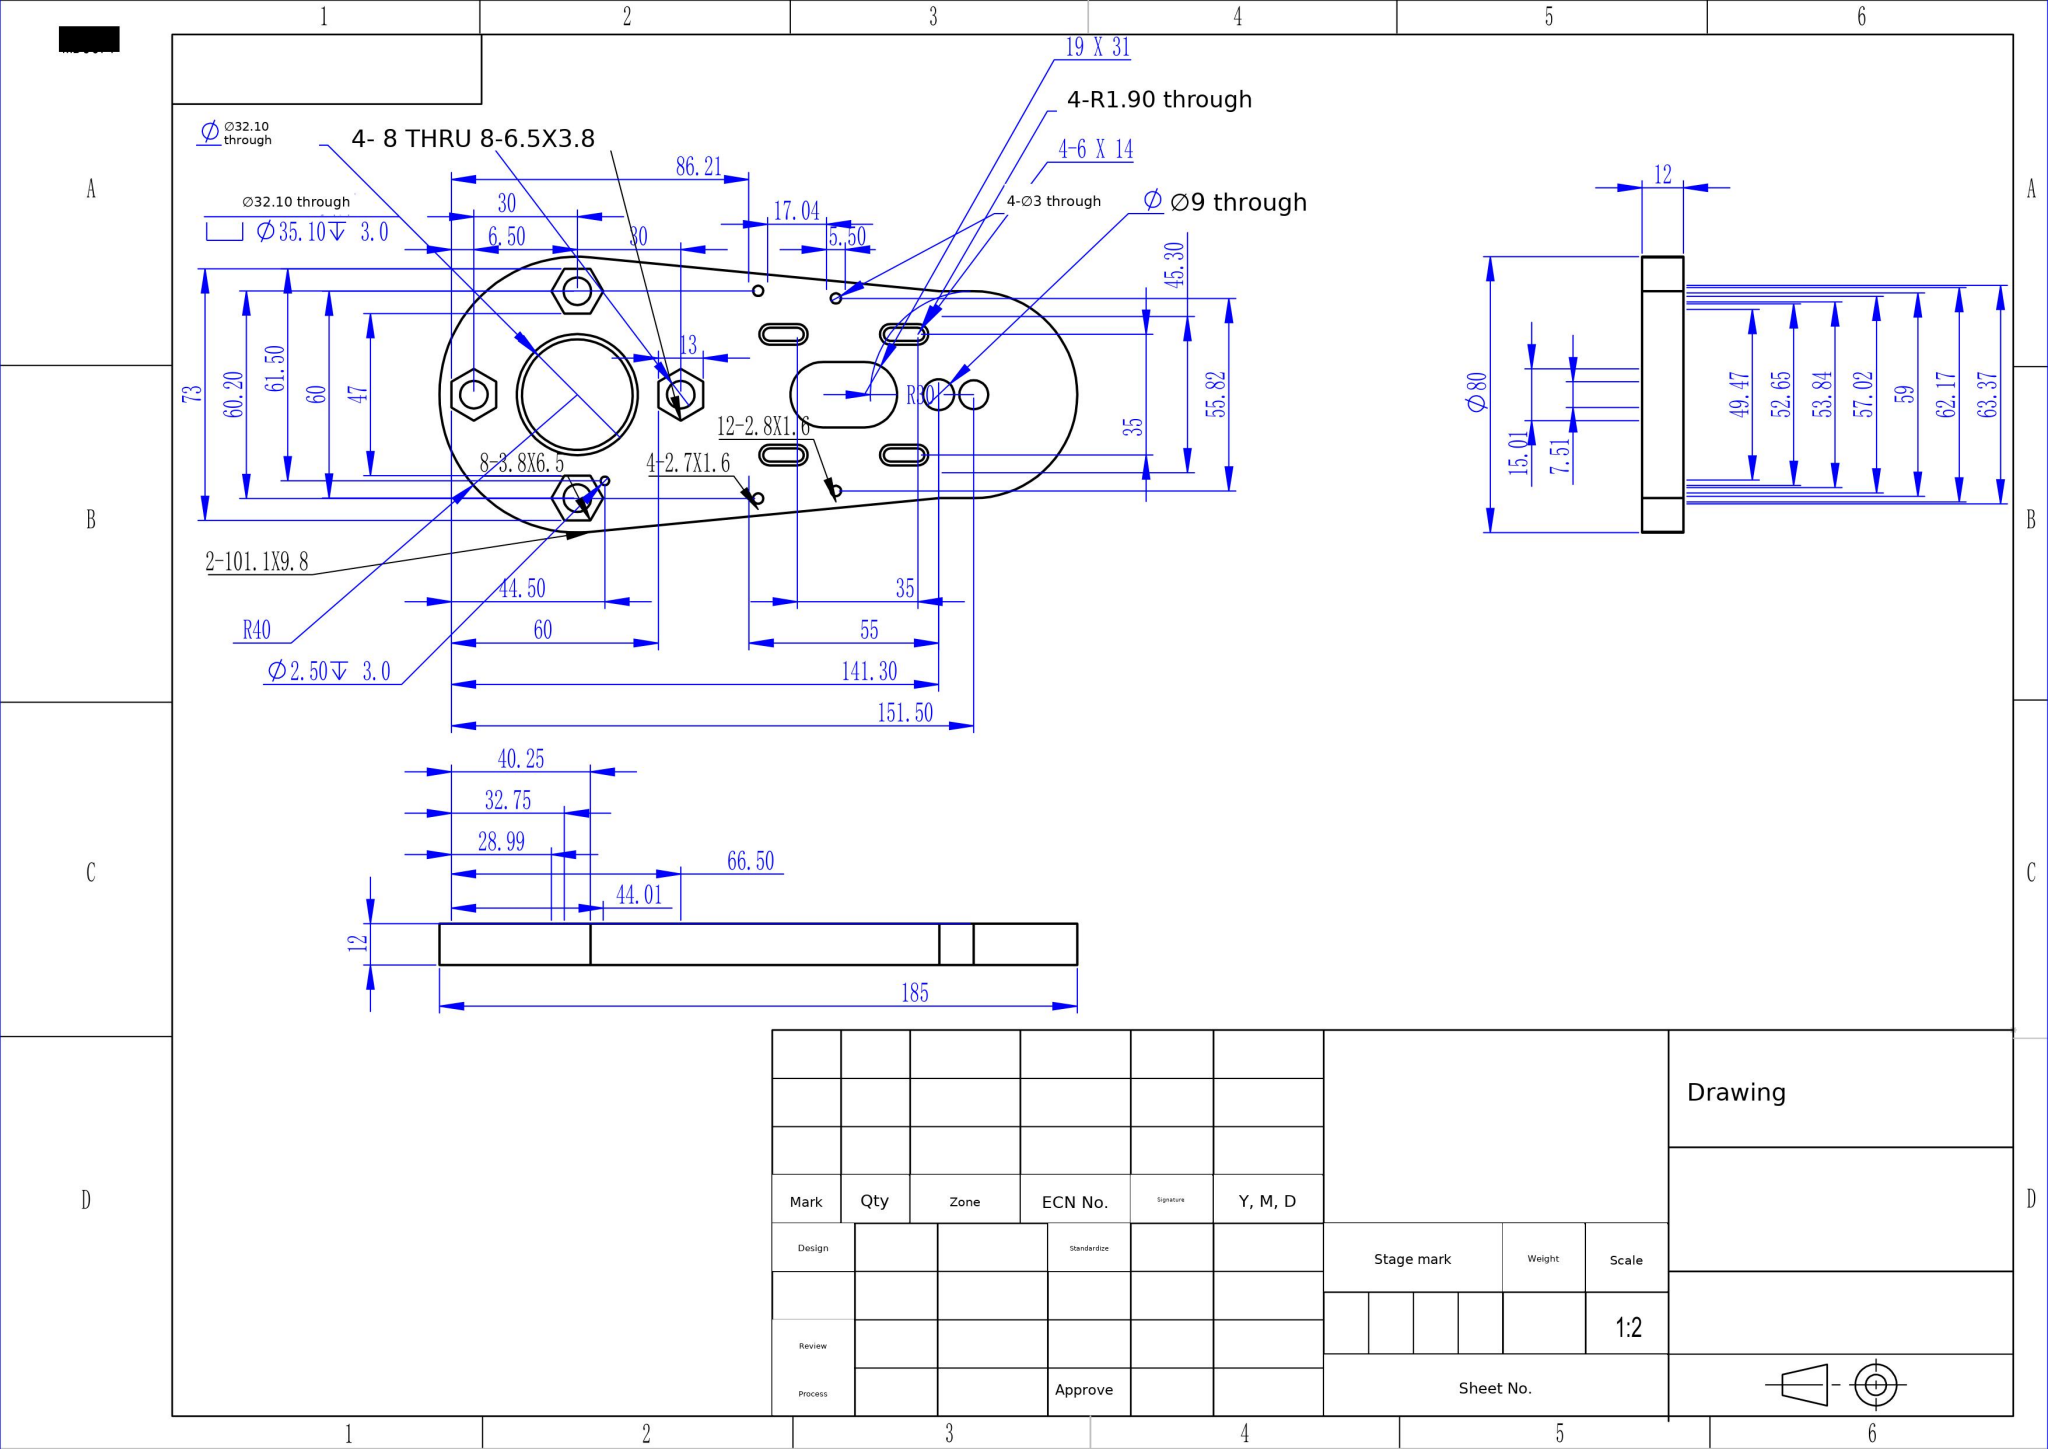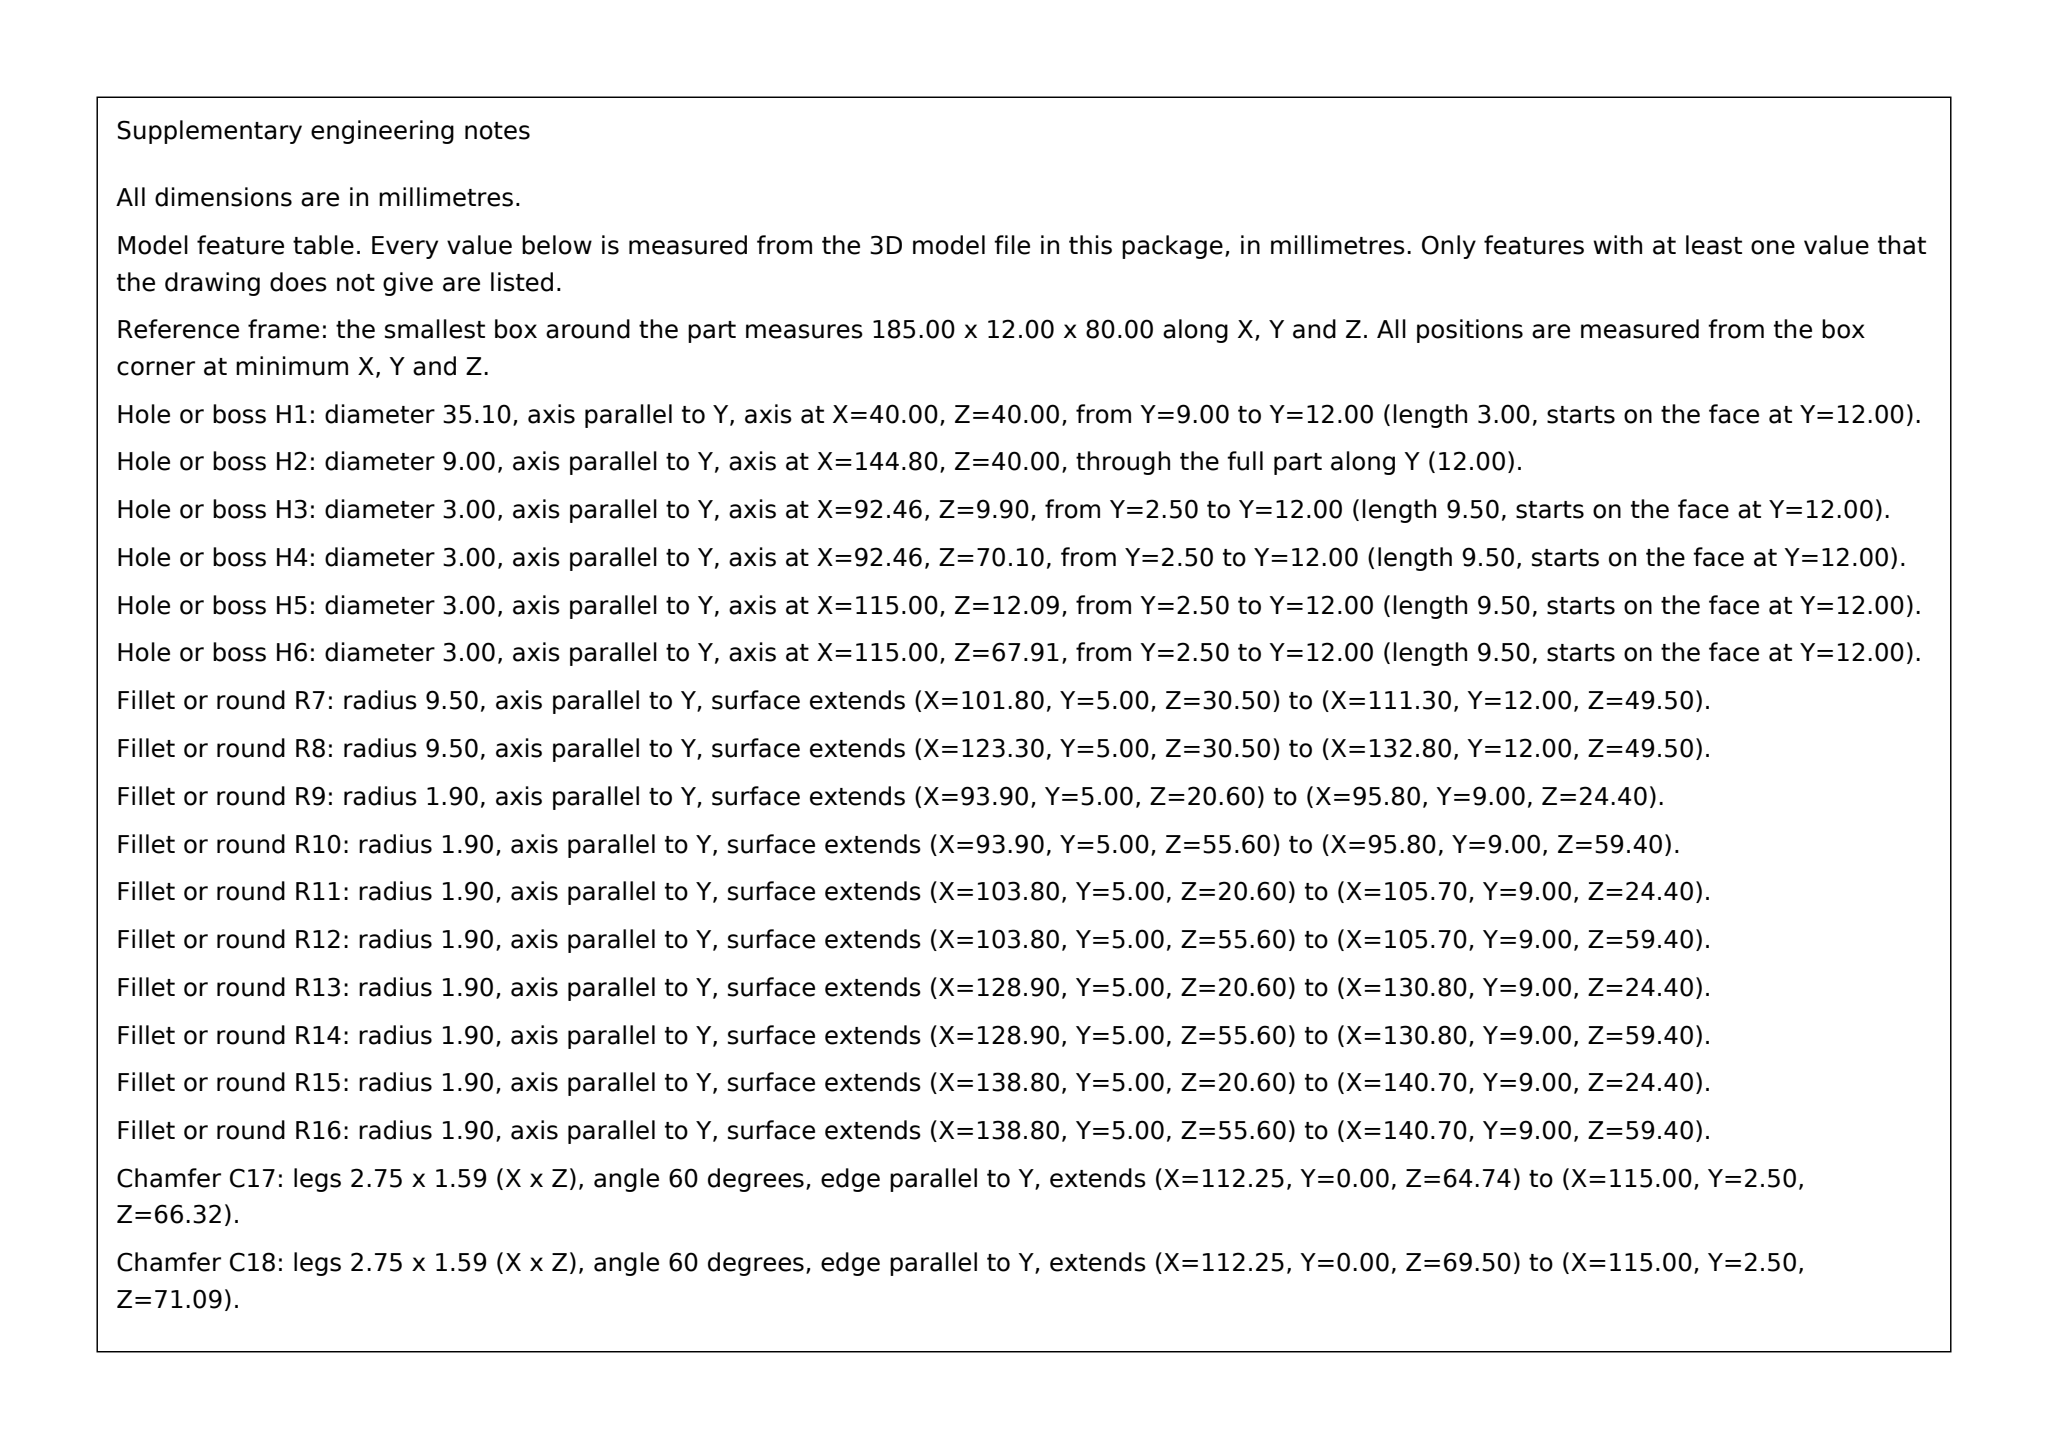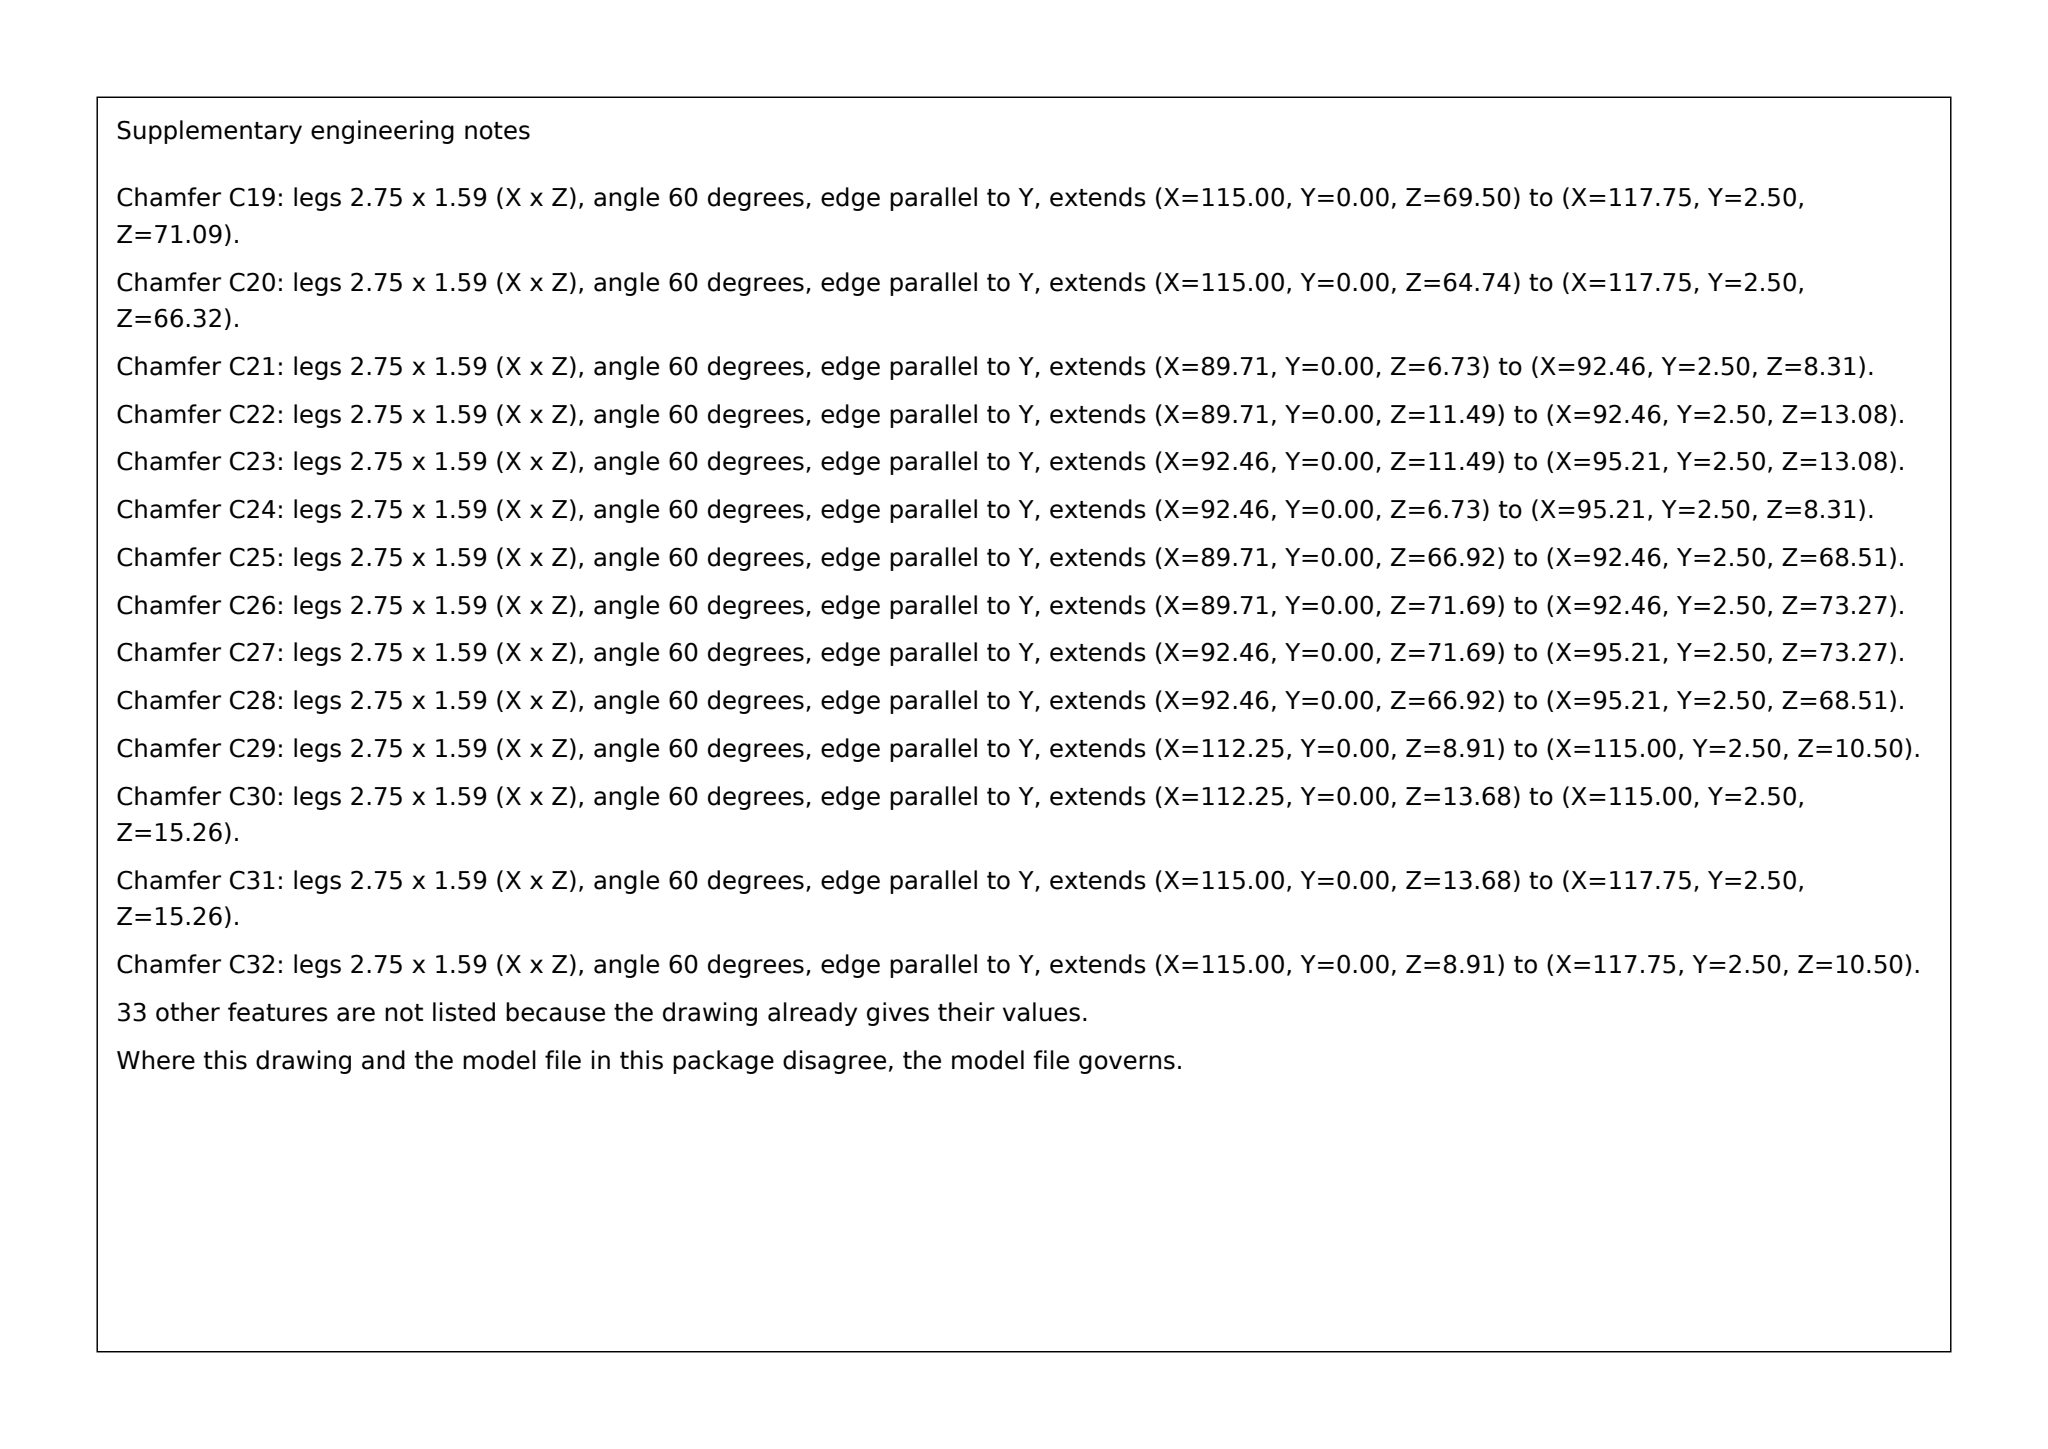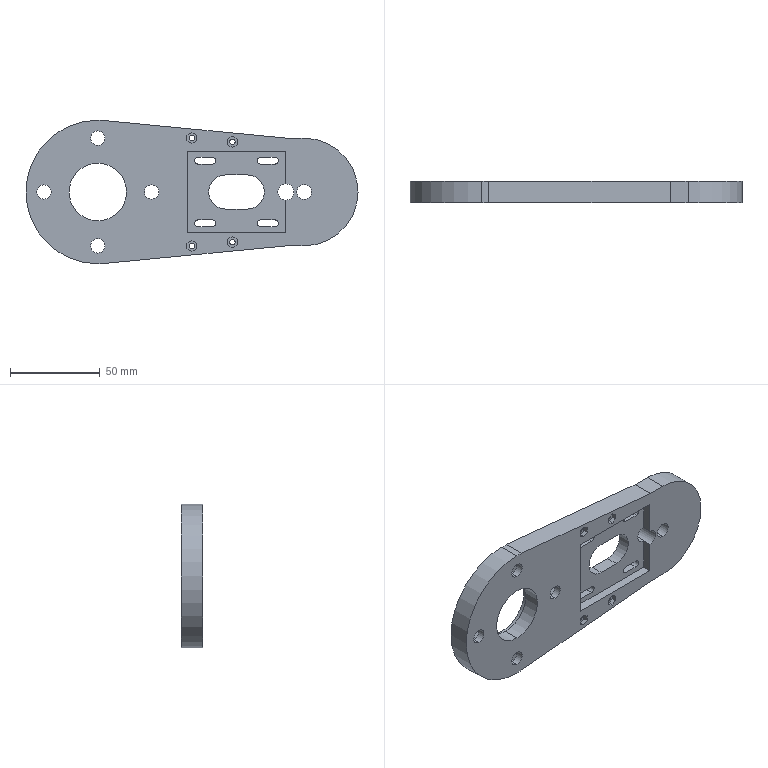Part | SolidWorks | mm | 1 solid | 140 faces | box 185 x 12 x 80 mm | volume 107645 mm3 | plane 92 | cylinder 48 | commonest cylinder face diameters 8 x8 3 x8 3.8 x8 6 x8 80 x3 2.5 x2 8.4 x2 32.1 x2
build123d program:
from build123d import *

# Parameters (mm, degrees)
SKETCH1_R            = 10
BOSS_EXTRUDE1_DEPTH  = 12
SKETCH2_R            = 17.55
CUT_EXTRUDE1_DEPTH   = 3
CUT_EXTRUDE2_DEPTH   = 12
SKETCH4_R            = 4
CUT_EXTRUDE3_DEPTH   = 12
SKETCH5_R            = 16.05
CUT_EXTRUDE4_DEPTH   = 113.721
CUT_EXTRUDE6_DEPTH   = 8
CUT_EXTRUDE7_DEPTH   = 3
SKETCH11_R           = 4.2
BOSS_EXTRUDE2_DEPTH  = 12
CUT_EXTRUDE1_2_DEPTH = 151.685
SKETCH1_2_R          = 4.5
CUT_EXTRUDE4_2_DEPTH = 151.894
SKETCH6_W            = 55
SKETCH6_H            = 45.3
CUT_EXTRUDE6_2_DEPTH = 5
SKETCH6_2_R          = 1.25
CUT_EXTRUDE9_DEPTH   = 3
SKETCH7_2_R          = 1.5
CUT_EXTRUDE10_DEPTH  = 151.894
CUT_EXTRUDE11_DEPTH  = 2.5


with BuildPart() as part:
    # Sketch1 → Boss-Extrude1 (new body)
    with BuildSketch(Plane(origin=(0, 0, 0), x_dir=(1, 0, 0), z_dir=(0, 1, 0))):
        with BuildLine():
            Line((3.863, 39.813), (105, 30))
            Line((105, 30), (105, -30))
            Line((105, -30), (3.863, -39.813))
            ThreePointArc((3.863, -39.813), (-40, 0), (3.863, 39.813))
        make_face()
        with Locations(Location((0, 0, 0), (0, 0, 270))):
            Circle(SKETCH1_R, mode=Mode.SUBTRACT)
    extrude(amount=BOSS_EXTRUDE1_DEPTH)

    # Sketch2 → Cut-Extrude1 (cut)
    with BuildSketch(Plane(origin=(0, 12, 0), x_dir=(1, 0, 0), z_dir=(0, 1, 0))):
        with Locations(Location((0, 0, 0), (0, 0, 270))):
            Circle(SKETCH2_R)
    extrude(amount=-CUT_EXTRUDE1_DEPTH, mode=Mode.SUBTRACT)

    # Sketch3 → Cut-Extrude2 (cut)
    with BuildSketch(Plane(origin=(0, 12, 0), x_dir=(1, 0, 0), z_dir=(0, 1, 0))):
        with BuildLine():
            Line((71.3, 9.5), (83.3, 9.5))
            ThreePointArc((83.3, 9.5), (92.8, 0), (83.3, -9.5))
            Line((83.3, -9.5), (71.3, -9.5))
            ThreePointArc((71.3, -9.5), (61.8, 0), (71.3, 9.5))
        make_face()
    extrude(amount=-CUT_EXTRUDE2_DEPTH, mode=Mode.SUBTRACT)

    # Sketch4 → Cut-Extrude3 (cut)
    with BuildSketch(Plane(origin=(0, 12, 0), x_dir=(1, 0, 0), z_dir=(0, 1, 0))):
        with Locations(Location((30, 0, 0), (0, 0, 270))):
            Circle(SKETCH4_R)
        with Locations(Location((0, -30, 0), (0, 0, 270))):
            Circle(SKETCH4_R)
        with Locations(Location((-30, 0, 0), (0, 0, 270))):
            Circle(SKETCH4_R)
        with Locations(Location((0, 30, 0), (0, 0, 270))):
            Circle(SKETCH4_R)
    extrude(amount=-CUT_EXTRUDE3_DEPTH, mode=Mode.SUBTRACT)

    # Sketch5 → Cut-Extrude4 (cut, through all)
    with BuildSketch(Plane.XZ.offset(-9)):
        with Locations(Location((0, 0, 0), (0, 0, 270))):
            Circle(SKETCH5_R)
    extrude(amount=CUT_EXTRUDE4_DEPTH, mode=Mode.SUBTRACT)

    # Sketch7 → Cut-Extrude6 (cut)
    with BuildSketch(Plane(origin=(0, 12, 0), x_dir=(1, 0, 0), z_dir=(0, 1, 0))):
        Polygon((-7.506, 30), (-3.753, 23.5), (3.753, 23.5), (7.506, 30), (3.753, 36.5), (-3.753, 36.5), align=None)
        Polygon((-30, -7.506), (-23.5, -3.753), (-23.5, 3.753), (-30, 7.506), (-36.5, 3.753), (-36.5, -3.753), align=None)
        Polygon((30, 7.506), (23.5, 3.753), (23.5, -3.753), (30, -7.506), (36.5, -3.753), (36.5, 3.753), align=None)
        Polygon((7.506, -30), (3.753, -23.5), (-3.753, -23.5), (-7.506, -30), (-3.753, -36.5), (3.753, -36.5), align=None)
    extrude(amount=-CUT_EXTRUDE6_DEPTH, mode=Mode.SUBTRACT)

    # Sketch9 → Cut-Extrude7 (cut)
    with BuildSketch(Plane(origin=(0, 12, 0), x_dir=(1, 0, 0), z_dir=(0, 1, 0))):
        with BuildLine():
            Line((55.8, 20.5), (63.8, 20.5))
            ThreePointArc((63.8, 20.5), (66.8, 17.5), (63.8, 14.5))
            Line((63.8, 14.5), (55.8, 14.5))
            ThreePointArc((55.8, 14.5), (52.8, 17.5), (55.8, 20.5))
        make_face()
        with BuildLine():
            Line((90.8, 20.5), (98.8, 20.5))
            ThreePointArc((98.8, 20.5), (101.8, 17.5), (98.8, 14.5))
            Line((98.8, 14.5), (90.8, 14.5))
            ThreePointArc((90.8, 14.5), (87.8, 17.5), (90.8, 20.5))
        make_face()
        with BuildLine():
            Line((55.8, -14.5), (63.8, -14.5))
            ThreePointArc((63.8, -14.5), (66.8, -17.5), (63.8, -20.5))
            Line((63.8, -20.5), (55.8, -20.5))
            ThreePointArc((55.8, -20.5), (52.8, -17.5), (55.8, -14.5))
        make_face()
        with BuildLine():
            Line((90.8, -14.5), (98.8, -14.5))
            ThreePointArc((98.8, -14.5), (101.8, -17.5), (98.8, -20.5))
            Line((98.8, -20.5), (90.8, -20.5))
            ThreePointArc((90.8, -20.5), (87.8, -17.5), (90.8, -14.5))
        make_face()
    extrude(amount=-CUT_EXTRUDE7_DEPTH, mode=Mode.SUBTRACT)

    # Sketch11 → Boss-Extrude2 (add)
    with BuildSketch(Plane(origin=(0, 12, 0), x_dir=(1, 0, 0), z_dir=(0, 1, 0))):
        with BuildLine():
            Line((105, -30), (105, 30))
            Line((105, 30), (115, 30))
            ThreePointArc((115, 30), (145, 0), (115, -30))
            Line((115, -30), (105, -30))
        make_face()
        with Locations(Location((115, 0, 0), (0, 0, 270))):
            Circle(SKETCH11_R, mode=Mode.SUBTRACT)
    extrude(amount=-BOSS_EXTRUDE2_DEPTH)

    # Sketch10 → Cut-Extrude1_2 (cut, through all)
    with BuildSketch(Plane(origin=(0, 9, 0), x_dir=(1, 0, 0), z_dir=(0, 1, 0))):
        with BuildLine():
            Line((55.8, 15.6), (63.8, 15.6))
            ThreePointArc((63.8, 15.6), (65.7, 17.5), (63.8, 19.4))
            Line((63.8, 19.4), (55.8, 19.4))
            ThreePointArc((55.8, 19.4), (53.9, 17.5), (55.8, 15.6))
        make_face()
        with BuildLine():
            Line((90.8, 15.6), (98.8, 15.6))
            ThreePointArc((98.8, 15.6), (100.7, 17.5), (98.8, 19.4))
            Line((98.8, 19.4), (90.8, 19.4))
            ThreePointArc((90.8, 19.4), (88.9, 17.5), (90.8, 15.6))
        make_face()
        with BuildLine():
            Line((55.8, -19.4), (63.8, -19.4))
            ThreePointArc((63.8, -19.4), (65.7, -17.5), (63.8, -15.6))
            Line((63.8, -15.6), (55.8, -15.6))
            ThreePointArc((55.8, -15.6), (53.9, -17.5), (55.8, -19.4))
        make_face()
        with BuildLine():
            Line((90.8, -19.4), (98.8, -19.4))
            ThreePointArc((98.8, -19.4), (100.7, -17.5), (98.8, -15.6))
            Line((98.8, -15.6), (90.8, -15.6))
            ThreePointArc((90.8, -15.6), (88.9, -17.5), (90.8, -19.4))
        make_face()
    extrude(amount=-CUT_EXTRUDE1_2_DEPTH, mode=Mode.SUBTRACT)

    # Sketch1_2 → Cut-Extrude4_2 (cut, through all)
    with BuildSketch(Plane(origin=(0, 12, 0), x_dir=(1, 0, 0), z_dir=(0, 1, 0))):
        with Locations(Location((104.8, 0, 0), (0, 0, 270))):
            Circle(SKETCH1_2_R)
    extrude(amount=-CUT_EXTRUDE4_2_DEPTH, mode=Mode.SUBTRACT)

    # Sketch6 → Cut-Extrude6_2 (cut)
    with BuildSketch(Plane.XZ):
        with Locations((77.3, 0)):
            Rectangle(SKETCH6_W, SKETCH6_H)
    extrude(amount=-CUT_EXTRUDE6_2_DEPTH, mode=Mode.SUBTRACT)

    # Sketch6_2 → Cut-Extrude9 (cut)
    with BuildSketch(Plane(origin=(0, 12, 0), x_dir=(1, 0, 0), z_dir=(0, 1, 0))):
        with Locations(Location((8, -25, 0), (0, 0, 270))):
            Circle(SKETCH6_2_R)
    extrude(amount=-CUT_EXTRUDE9_DEPTH, mode=Mode.SUBTRACT)

    # Sketch7_2 → Cut-Extrude10 (cut, through all)
    with BuildSketch(Plane.XZ):
        with Locations(Location((75, -27.911, 0), (0, 0, 270))):
            Circle(SKETCH7_2_R)
        with Locations(Location((75, 27.911, 0), (0, 0, 270))):
            Circle(SKETCH7_2_R)
        with Locations(Location((52.46, -30.098, 0), (0, 0, 270))):
            Circle(SKETCH7_2_R)
        with Locations(Location((52.46, 30.098, 0), (0, 0, 270))):
            Circle(SKETCH7_2_R)
    extrude(amount=-CUT_EXTRUDE10_DEPTH, mode=Mode.SUBTRACT)

    # Sketch4_2 → Cut-Extrude11 (cut)
    with BuildSketch(Plane.XZ):
        Polygon((75, 24.735), (77.75, 26.323), (77.75, 29.499), (75, 31.086), (72.25, 29.499), (72.25, 26.323), align=None)
        Polygon((75, -31.086), (77.75, -29.499), (77.75, -26.323), (75, -24.735), (72.25, -26.323), (72.25, -29.499), align=None)
        Polygon((52.46, 26.922), (55.21, 28.51), (55.21, 31.685), (52.46, 33.273), (49.71, 31.685), (49.71, 28.51), align=None)
        Polygon((52.46, -33.273), (55.21, -31.685), (55.21, -28.51), (52.46, -26.922), (49.71, -28.51), (49.71, -31.685), align=None)
    extrude(amount=-CUT_EXTRUDE11_DEPTH, mode=Mode.SUBTRACT)


solid = part.part